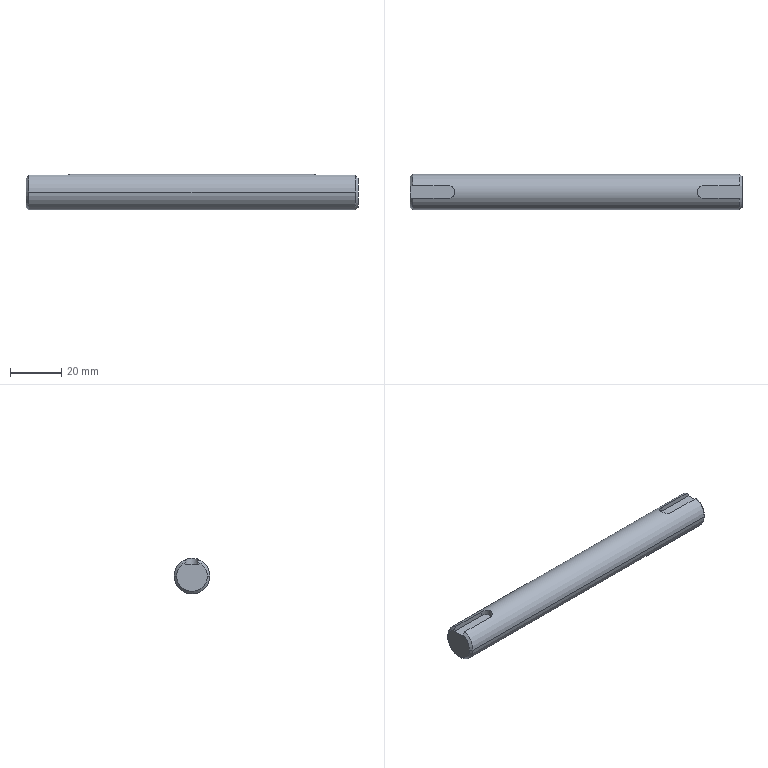Component | SolidWorks | DriveAxis-1 | 1 solid | 18 faces | box 130 x 14 x 14 mm | volume 19610 mm3 | plane 8 | cone 6 | cylinder 4 | commonest cylinder face diameters 14 x2 5 x2
build123d program:
from build123d import *

# Parameters (mm, degrees)
SKETCH1_R           = 7
BOSS_EXTRUDE1_DEPTH = 130
CHAMFER1_SIZE       = 1
CUT_EXTRUDE1_DEPTH  = 2.3


with BuildPart() as part:
    # Sketch1 → Boss-Extrude1 (new body)
    with BuildSketch(Plane(origin=(0, 0, 0), x_dir=(1, 0, 0), z_dir=(0, 1, 0))):
        with Locations(Location((0, 0, 0), (0, 0, 270))):
            Circle(SKETCH1_R)
    extrude(amount=BOSS_EXTRUDE1_DEPTH)

    # Chamfer1
    chamfer1_edges = [part.edges().sort_by_distance(p)[0] for p in [
        (0, 0, -7),
        (0, 130, -7),
    ]]
    chamfer(chamfer1_edges, length=CHAMFER1_SIZE)

    # Sketch2 → Cut-Extrude1 (cut)
    with BuildSketch(Plane.ZY.offset(7)):
        with BuildLine():
            Line((-2.5, 0), (-2.5, 15))
            ThreePointArc((-2.5, 15), (0, 17.5), (2.5, 15))
            Line((2.5, 15), (2.5, 0))
            ThreePointArc((2.5, 0), (0, -2.5), (-2.5, 0))
        make_face()
    cut_extrude1 = extrude(amount=-CUT_EXTRUDE1_DEPTH, mode=Mode.SUBTRACT)

    # Mirror1: Cut-Extrude1 across plane
    add(cut_extrude1.mirror(Plane(origin=(0, 65, 0), x_dir=(0, 0, 1), z_dir=(0, -1, 0))), mode=Mode.SUBTRACT)


solid = part.part

# Placed as in the assembly
solid = solid.moved(Location((15.629, -347.9, 460), (90, 0, -90)))
STEP:
#1=COLOUR_RGB('',0.7922,0.8196,0.9333);
#2=FILL_AREA_STYLE_COLOUR('',#1);
#3=FILL_AREA_STYLE('',(#2));
#4=SURFACE_STYLE_FILL_AREA(#3);
#5=SURFACE_SIDE_STYLE('',(#4));
#6=SURFACE_STYLE_USAGE(.BOTH.,#5);
#7=PRESENTATION_STYLE_ASSIGNMENT((#6));
#8=CARTESIAN_POINT('',(0.6153,-13.461,18.11));
#9=VERTEX_POINT('',#8);
#10=CARTESIAN_POINT('',(0.6153,-13.933,18.11));
#11=VERTEX_POINT('',#10);
#12=CARTESIAN_POINT('',(0.6153,-13.697,18.11));
#13=DIRECTION('',(-1.,0.,0.));
#14=DIRECTION('',(0.,-1.,0.));
#15=AXIS2_PLACEMENT_3D('',#12,#13,#14);
#16=CIRCLE('',#15,0.2362);
#17=EDGE_CURVE('',#9,#11,#16,.T.);
#18=ORIENTED_EDGE('',*,*,#17,.F.);
#19=CARTESIAN_POINT('',(0.6547,-13.421,18.11));
#20=VERTEX_POINT('',#19);
#21=CARTESIAN_POINT('',(0.6547,-13.421,18.11));
#22=DIRECTION('',(0.7071,0.7071,0.));
#23=VECTOR('',#22,39.37);
#24=LINE('',#21,#23);
#25=EDGE_CURVE('',#9,#20,#24,.T.);
#26=ORIENTED_EDGE('',*,*,#25,.T.);
#27=CARTESIAN_POINT('',(0.6547,-13.972,18.11));
#28=VERTEX_POINT('',#27);
#29=CARTESIAN_POINT('',(0.6547,-13.697,18.11));
#30=DIRECTION('',(1.,-0.,-0.));
#31=DIRECTION('',(0.,-1.,0.));
#32=AXIS2_PLACEMENT_3D('',#29,#30,#31);
#33=CIRCLE('',#32,0.2756);
#34=EDGE_CURVE('',#28,#20,#33,.T.);
#35=ORIENTED_EDGE('',*,*,#34,.F.);
#36=CARTESIAN_POINT('',(0.6547,-13.972,18.11));
#37=DIRECTION('',(0.7071,-0.7071,-0.));
#38=VECTOR('',#37,39.37);
#39=LINE('',#36,#38);
#40=EDGE_CURVE('',#11,#28,#39,.T.);
#41=ORIENTED_EDGE('',*,*,#40,.F.);
#42=EDGE_LOOP('',(#18,#26,#35,#41));
#43=FACE_OUTER_BOUND('',#42,.T.);
#44=CARTESIAN_POINT('',(0.6547,-13.697,18.11));
#45=DIRECTION('',(1.,-0.,-0.));
#46=DIRECTION('',(0.,-1.,0.));
#47=AXIS2_PLACEMENT_3D('',#44,#45,#46);
#48=CONICAL_SURFACE('',#47,0.2756,0.7854);
#49=ADVANCED_FACE('',(#43),#48,.T.);
#50=CARTESIAN_POINT('',(0.6153,-13.795,18.325));
#51=VERTEX_POINT('',#50);
#52=CARTESIAN_POINT('',(0.6153,-13.697,18.11));
#53=DIRECTION('',(-1.,0.,0.));
#54=DIRECTION('',(0.,-1.,0.));
#55=AXIS2_PLACEMENT_3D('',#52,#53,#54);
#56=CIRCLE('',#55,0.2362);
#57=EDGE_CURVE('',#11,#51,#56,.T.);
#58=ORIENTED_EDGE('',*,*,#57,.F.);
#59=ORIENTED_EDGE('',*,*,#40,.T.);
#60=CARTESIAN_POINT('',(0.6547,-13.795,18.368));
#61=VERTEX_POINT('',#60);
#62=CARTESIAN_POINT('',(0.6547,-13.697,18.11));
#63=DIRECTION('',(1.,-0.,-0.));
#64=DIRECTION('',(0.,-1.,0.));
#65=AXIS2_PLACEMENT_3D('',#62,#63,#64);
#66=CIRCLE('',#65,0.2756);
#67=EDGE_CURVE('',#61,#28,#66,.T.);
#68=ORIENTED_EDGE('',*,*,#67,.F.);
#69=CARTESIAN_POINT('',(0.6153,-13.795,18.325));
#70=CARTESIAN_POINT('',(0.6283,-13.795,18.339));
#71=CARTESIAN_POINT('',(0.6415,-13.795,18.354));
#72=CARTESIAN_POINT('',(0.6547,-13.795,18.368));
#73=B_SPLINE_CURVE_WITH_KNOTS('',3,(#69,#70,#71,#72),.UNSPECIFIED.,.F.,.F.,(4,4),(0.003923,0.005397),.UNSPECIFIED.);
#74=EDGE_CURVE('',#51,#61,#73,.T.);
#75=ORIENTED_EDGE('',*,*,#74,.F.);
#76=EDGE_LOOP('',(#58,#59,#68,#75));
#77=FACE_OUTER_BOUND('',#76,.T.);
#78=CARTESIAN_POINT('',(0.6547,-13.697,18.11));
#79=DIRECTION('',(1.,-0.,-0.));
#80=DIRECTION('',(0.,-1.,0.));
#81=AXIS2_PLACEMENT_3D('',#78,#79,#80);
#82=CONICAL_SURFACE('',#81,0.2756,0.7854);
#83=ADVANCED_FACE('',(#77),#82,.T.);
#84=CARTESIAN_POINT('',(5.733,-13.933,18.11));
#85=VERTEX_POINT('',#84);
#86=CARTESIAN_POINT('',(5.733,-13.461,18.11));
#87=VERTEX_POINT('',#86);
#88=CARTESIAN_POINT('',(5.733,-13.697,18.11));
#89=DIRECTION('',(1.,-0.,-0.));
#90=DIRECTION('',(0.,-1.,0.));
#91=AXIS2_PLACEMENT_3D('',#88,#89,#90);
#92=CIRCLE('',#91,0.2362);
#93=EDGE_CURVE('',#85,#87,#92,.T.);
#94=ORIENTED_EDGE('',*,*,#93,.F.);
#95=CARTESIAN_POINT('',(5.694,-13.972,18.11));
#96=VERTEX_POINT('',#95);
#97=CARTESIAN_POINT('',(5.733,-13.933,18.11));
#98=DIRECTION('',(-0.7071,-0.7071,-0.));
#99=VECTOR('',#98,39.37);
#100=LINE('',#97,#99);
#101=EDGE_CURVE('',#85,#96,#100,.T.);
#102=ORIENTED_EDGE('',*,*,#101,.T.);
#103=CARTESIAN_POINT('',(5.694,-13.421,18.11));
#104=VERTEX_POINT('',#103);
#105=CARTESIAN_POINT('',(5.694,-13.697,18.11));
#106=DIRECTION('',(-1.,0.,0.));
#107=DIRECTION('',(0.,-1.,-0.));
#108=AXIS2_PLACEMENT_3D('',#105,#106,#107);
#109=CIRCLE('',#108,0.2756);
#110=EDGE_CURVE('',#104,#96,#109,.T.);
#111=ORIENTED_EDGE('',*,*,#110,.F.);
#112=CARTESIAN_POINT('',(5.733,-13.461,18.11));
#113=DIRECTION('',(-0.7071,0.7071,0.));
#114=VECTOR('',#113,39.37);
#115=LINE('',#112,#114);
#116=EDGE_CURVE('',#87,#104,#115,.T.);
#117=ORIENTED_EDGE('',*,*,#116,.F.);
#118=EDGE_LOOP('',(#94,#102,#111,#117));
#119=FACE_OUTER_BOUND('',#118,.T.);
#120=CARTESIAN_POINT('',(5.733,-13.697,18.11));
#121=DIRECTION('',(-1.,0.,0.));
#122=DIRECTION('',(0.,1.,0.));
#123=AXIS2_PLACEMENT_3D('',#120,#121,#122);
#124=CONICAL_SURFACE('',#123,0.2362,0.7854);
#125=ADVANCED_FACE('',(#119),#124,.T.);
#126=CARTESIAN_POINT('',(5.733,-13.598,18.325));
#127=VERTEX_POINT('',#126);
#128=CARTESIAN_POINT('',(5.733,-13.697,18.11));
#129=DIRECTION('',(1.,-0.,-0.));
#130=DIRECTION('',(0.,-1.,0.));
#131=AXIS2_PLACEMENT_3D('',#128,#129,#130);
#132=CIRCLE('',#131,0.2362);
#133=EDGE_CURVE('',#87,#127,#132,.T.);
#134=ORIENTED_EDGE('',*,*,#133,.F.);
#135=ORIENTED_EDGE('',*,*,#116,.T.);
#136=CARTESIAN_POINT('',(5.694,-13.598,18.368));
#137=VERTEX_POINT('',#136);
#138=CARTESIAN_POINT('',(5.694,-13.697,18.11));
#139=DIRECTION('',(-1.,0.,0.));
#140=DIRECTION('',(0.,-1.,-0.));
#141=AXIS2_PLACEMENT_3D('',#138,#139,#140);
#142=CIRCLE('',#141,0.2756);
#143=EDGE_CURVE('',#137,#104,#142,.T.);
#144=ORIENTED_EDGE('',*,*,#143,.F.);
#145=CARTESIAN_POINT('',(5.694,-13.598,18.368));
#146=CARTESIAN_POINT('',(5.707,-13.598,18.354));
#147=CARTESIAN_POINT('',(5.72,-13.598,18.339));
#148=CARTESIAN_POINT('',(5.733,-13.598,18.325));
#149=B_SPLINE_CURVE_WITH_KNOTS('',3,(#145,#146,#147,#148),.UNSPECIFIED.,.F.,.F.,(4,4),(0.003636,0.005111),.UNSPECIFIED.);
#150=EDGE_CURVE('',#137,#127,#149,.T.);
#151=ORIENTED_EDGE('',*,*,#150,.T.);
#152=EDGE_LOOP('',(#134,#135,#144,#151));
#153=FACE_OUTER_BOUND('',#152,.T.);
#154=CARTESIAN_POINT('',(5.733,-13.697,18.11));
#155=DIRECTION('',(-1.,0.,0.));
#156=DIRECTION('',(0.,1.,0.));
#157=AXIS2_PLACEMENT_3D('',#154,#155,#156);
#158=CONICAL_SURFACE('',#157,0.2362,0.7854);
#159=ADVANCED_FACE('',(#153),#158,.T.);
#160=ORIENTED_EDGE('',*,*,#110,.T.);
#161=CARTESIAN_POINT('',(5.733,-13.972,18.11));
#162=DIRECTION('',(-1.,0.,0.));
#163=VECTOR('',#162,39.37);
#164=LINE('',#161,#163);
#165=EDGE_CURVE('',#96,#28,#164,.T.);
#166=ORIENTED_EDGE('',*,*,#165,.T.);
#167=ORIENTED_EDGE('',*,*,#34,.T.);
#168=CARTESIAN_POINT('',(5.733,-13.421,18.11));
#169=DIRECTION('',(-1.,0.,0.));
#170=VECTOR('',#169,39.37);
#171=LINE('',#168,#170);
#172=EDGE_CURVE('',#104,#20,#171,.T.);
#173=ORIENTED_EDGE('',*,*,#172,.F.);
#174=EDGE_LOOP('',(#160,#166,#167,#173));
#175=FACE_OUTER_BOUND('',#174,.T.);
#176=CARTESIAN_POINT('',(5.733,-13.697,18.11));
#177=DIRECTION('',(-1.,0.,0.));
#178=DIRECTION('',(0.,1.,0.));
#179=AXIS2_PLACEMENT_3D('',#176,#177,#178);
#180=CYLINDRICAL_SURFACE('',#179,0.2756);
#181=ADVANCED_FACE('',(#175),#180,.T.);
#182=ORIENTED_EDGE('',*,*,#165,.F.);
#183=CARTESIAN_POINT('',(5.694,-13.795,18.368));
#184=VERTEX_POINT('',#183);
#185=CARTESIAN_POINT('',(5.694,-13.697,18.11));
#186=DIRECTION('',(-1.,0.,0.));
#187=DIRECTION('',(0.,-1.,0.));
#188=AXIS2_PLACEMENT_3D('',#185,#186,#187);
#189=CIRCLE('',#188,0.2756);
#190=EDGE_CURVE('',#96,#184,#189,.T.);
#191=ORIENTED_EDGE('',*,*,#190,.T.);
#192=CARTESIAN_POINT('',(5.143,-13.795,18.368));
#193=VERTEX_POINT('',#192);
#194=CARTESIAN_POINT('',(5.733,-13.795,18.368));
#195=DIRECTION('',(1.,-0.,-0.));
#196=VECTOR('',#195,39.37);
#197=LINE('',#194,#196);
#198=EDGE_CURVE('',#193,#184,#197,.T.);
#199=ORIENTED_EDGE('',*,*,#198,.F.);
#200=CARTESIAN_POINT('',(5.143,-13.598,18.368));
#201=VERTEX_POINT('',#200);
#202=CARTESIAN_POINT('',(5.143,-13.598,18.368));
#203=CARTESIAN_POINT('',(5.136,-13.598,18.368));
#204=CARTESIAN_POINT('',(5.13,-13.599,18.368));
#205=CARTESIAN_POINT('',(5.117,-13.602,18.369));
#206=CARTESIAN_POINT('',(5.111,-13.604,18.37));
#207=CARTESIAN_POINT('',(5.099,-13.608,18.371));
#208=CARTESIAN_POINT('',(5.093,-13.612,18.372));
#209=CARTESIAN_POINT('',(5.083,-13.619,18.375));
#210=CARTESIAN_POINT('',(5.078,-13.623,18.376));
#211=CARTESIAN_POINT('',(5.064,-13.636,18.379));
#212=CARTESIAN_POINT('',(5.057,-13.647,18.382));
#213=CARTESIAN_POINT('',(5.05,-13.665,18.384));
#214=CARTESIAN_POINT('',(5.048,-13.671,18.385));
#215=CARTESIAN_POINT('',(5.045,-13.684,18.386));
#216=CARTESIAN_POINT('',(5.044,-13.69,18.386));
#217=CARTESIAN_POINT('',(5.044,-13.703,18.386));
#218=CARTESIAN_POINT('',(5.045,-13.71,18.386));
#219=CARTESIAN_POINT('',(5.048,-13.722,18.385));
#220=CARTESIAN_POINT('',(5.05,-13.729,18.384));
#221=CARTESIAN_POINT('',(5.054,-13.741,18.382));
#222=CARTESIAN_POINT('',(5.058,-13.746,18.381));
#223=CARTESIAN_POINT('',(5.065,-13.757,18.379));
#224=CARTESIAN_POINT('',(5.069,-13.762,18.378));
#225=CARTESIAN_POINT('',(5.078,-13.771,18.376));
#226=CARTESIAN_POINT('',(5.083,-13.775,18.375));
#227=CARTESIAN_POINT('',(5.093,-13.782,18.372));
#228=CARTESIAN_POINT('',(5.099,-13.785,18.371));
#229=CARTESIAN_POINT('',(5.111,-13.79,18.37));
#230=CARTESIAN_POINT('',(5.117,-13.792,18.369));
#231=CARTESIAN_POINT('',(5.13,-13.795,18.368));
#232=CARTESIAN_POINT('',(5.136,-13.795,18.368));
#233=CARTESIAN_POINT('',(5.143,-13.795,18.368));
#234=B_SPLINE_CURVE_WITH_KNOTS('',3,(#202,#203,#204,#205,#206,#207,#208,#209,#210,#211,#212,#213,#214,#215,#216,#217,#218,#219,#220,#221,#222,#223,#224,#225,#226,#227,#228,#229,#230,#231,#232,#233),.UNSPECIFIED.,.F.,.F.,(4,2,2,2,2,2,2,2,2,2,2,2,2,2,2,4),(0.,0.0004924,0.0009848,0.001477,0.00197,0.002954,0.003447,0.003939,0.004432,0.004924,0.005416,0.005909,0.006401,0.006894,0.007386,0.007878),.UNSPECIFIED.);
#235=EDGE_CURVE('',#201,#193,#234,.T.);
#236=ORIENTED_EDGE('',*,*,#235,.F.);
#237=CARTESIAN_POINT('',(5.733,-13.598,18.368));
#238=DIRECTION('',(-1.,0.,0.));
#239=VECTOR('',#238,39.37);
#240=LINE('',#237,#239);
#241=EDGE_CURVE('',#137,#201,#240,.T.);
#242=ORIENTED_EDGE('',*,*,#241,.F.);
#243=ORIENTED_EDGE('',*,*,#143,.T.);
#244=ORIENTED_EDGE('',*,*,#172,.T.);
#245=CARTESIAN_POINT('',(0.6547,-13.598,18.368));
#246=VERTEX_POINT('',#245);
#247=CARTESIAN_POINT('',(0.6547,-13.697,18.11));
#248=DIRECTION('',(1.,-0.,-0.));
#249=DIRECTION('',(0.,-1.,0.));
#250=AXIS2_PLACEMENT_3D('',#247,#248,#249);
#251=CIRCLE('',#250,0.2756);
#252=EDGE_CURVE('',#20,#246,#251,.T.);
#253=ORIENTED_EDGE('',*,*,#252,.T.);
#254=CARTESIAN_POINT('',(1.206,-13.598,18.368));
#255=VERTEX_POINT('',#254);
#256=CARTESIAN_POINT('',(5.733,-13.598,18.368));
#257=DIRECTION('',(1.,-0.,-0.));
#258=VECTOR('',#257,39.37);
#259=LINE('',#256,#258);
#260=EDGE_CURVE('',#246,#255,#259,.T.);
#261=ORIENTED_EDGE('',*,*,#260,.T.);
#262=CARTESIAN_POINT('',(1.206,-13.795,18.368));
#263=VERTEX_POINT('',#262);
#264=CARTESIAN_POINT('',(1.206,-13.598,18.368));
#265=CARTESIAN_POINT('',(1.212,-13.598,18.368));
#266=CARTESIAN_POINT('',(1.219,-13.599,18.368));
#267=CARTESIAN_POINT('',(1.232,-13.602,18.369));
#268=CARTESIAN_POINT('',(1.238,-13.604,18.37));
#269=CARTESIAN_POINT('',(1.25,-13.608,18.371));
#270=CARTESIAN_POINT('',(1.255,-13.612,18.372));
#271=CARTESIAN_POINT('',(1.266,-13.619,18.375));
#272=CARTESIAN_POINT('',(1.271,-13.623,18.376));
#273=CARTESIAN_POINT('',(1.284,-13.636,18.379));
#274=CARTESIAN_POINT('',(1.292,-13.647,18.382));
#275=CARTESIAN_POINT('',(1.299,-13.665,18.384));
#276=CARTESIAN_POINT('',(1.301,-13.671,18.385));
#277=CARTESIAN_POINT('',(1.304,-13.684,18.386));
#278=CARTESIAN_POINT('',(1.304,-13.69,18.386));
#279=CARTESIAN_POINT('',(1.304,-13.703,18.386));
#280=CARTESIAN_POINT('',(1.304,-13.71,18.386));
#281=CARTESIAN_POINT('',(1.301,-13.722,18.385));
#282=CARTESIAN_POINT('',(1.299,-13.729,18.384));
#283=CARTESIAN_POINT('',(1.294,-13.741,18.382));
#284=CARTESIAN_POINT('',(1.291,-13.746,18.381));
#285=CARTESIAN_POINT('',(1.284,-13.757,18.379));
#286=CARTESIAN_POINT('',(1.28,-13.762,18.378));
#287=CARTESIAN_POINT('',(1.271,-13.771,18.376));
#288=CARTESIAN_POINT('',(1.266,-13.775,18.375));
#289=CARTESIAN_POINT('',(1.255,-13.782,18.372));
#290=CARTESIAN_POINT('',(1.25,-13.785,18.371));
#291=CARTESIAN_POINT('',(1.238,-13.79,18.37));
#292=CARTESIAN_POINT('',(1.232,-13.792,18.369));
#293=CARTESIAN_POINT('',(1.219,-13.795,18.368));
#294=CARTESIAN_POINT('',(1.212,-13.795,18.368));
#295=CARTESIAN_POINT('',(1.206,-13.795,18.368));
#296=B_SPLINE_CURVE_WITH_KNOTS('',3,(#264,#265,#266,#267,#268,#269,#270,#271,#272,#273,#274,#275,#276,#277,#278,#279,#280,#281,#282,#283,#284,#285,#286,#287,#288,#289,#290,#291,#292,#293,#294,#295),.UNSPECIFIED.,.F.,.F.,(4,2,2,2,2,2,2,2,2,2,2,2,2,2,2,4),(0.,0.0004924,0.0009848,0.001477,0.00197,0.002954,0.003447,0.003939,0.004432,0.004924,0.005416,0.005909,0.006401,0.006894,0.007386,0.007878),.UNSPECIFIED.);
#297=EDGE_CURVE('',#255,#263,#296,.T.);
#298=ORIENTED_EDGE('',*,*,#297,.T.);
#299=CARTESIAN_POINT('',(5.733,-13.795,18.368));
#300=DIRECTION('',(-1.,0.,0.));
#301=VECTOR('',#300,39.37);
#302=LINE('',#299,#301);
#303=EDGE_CURVE('',#263,#61,#302,.T.);
#304=ORIENTED_EDGE('',*,*,#303,.T.);
#305=ORIENTED_EDGE('',*,*,#67,.T.);
#306=EDGE_LOOP('',(#182,#191,#199,#236,#242,#243,#244,#253,#261,#298,#304,#305));
#307=FACE_OUTER_BOUND('',#306,.T.);
#308=CARTESIAN_POINT('',(5.733,-13.697,18.11));
#309=DIRECTION('',(-1.,0.,0.));
#310=DIRECTION('',(0.,1.,0.));
#311=AXIS2_PLACEMENT_3D('',#308,#309,#310);
#312=CYLINDRICAL_SURFACE('',#311,0.2756);
#313=ADVANCED_FACE('',(#307),#312,.T.);
#314=CARTESIAN_POINT('',(5.733,-13.598,18.295));
#315=VERTEX_POINT('',#314);
#316=CARTESIAN_POINT('',(5.733,-13.795,18.295));
#317=VERTEX_POINT('',#316);
#318=CARTESIAN_POINT('',(5.733,-13.697,18.295));
#319=DIRECTION('',(-0.,-1.,-0.));
#320=VECTOR('',#319,39.37);
#321=LINE('',#318,#320);
#322=EDGE_CURVE('',#315,#317,#321,.T.);
#323=ORIENTED_EDGE('',*,*,#322,.T.);
#324=CARTESIAN_POINT('',(5.733,-13.795,18.325));
#325=VERTEX_POINT('',#324);
#326=CARTESIAN_POINT('',(5.733,-13.795,18.295));
#327=DIRECTION('',(0.,-0.,1.));
#328=VECTOR('',#327,39.37);
#329=LINE('',#326,#328);
#330=EDGE_CURVE('',#317,#325,#329,.T.);
#331=ORIENTED_EDGE('',*,*,#330,.T.);
#332=CARTESIAN_POINT('',(5.733,-13.697,18.11));
#333=DIRECTION('',(1.,-0.,-0.));
#334=DIRECTION('',(0.,-1.,0.));
#335=AXIS2_PLACEMENT_3D('',#332,#333,#334);
#336=CIRCLE('',#335,0.2362);
#337=EDGE_CURVE('',#325,#85,#336,.T.);
#338=ORIENTED_EDGE('',*,*,#337,.T.);
#339=ORIENTED_EDGE('',*,*,#93,.T.);
#340=ORIENTED_EDGE('',*,*,#133,.T.);
#341=CARTESIAN_POINT('',(5.733,-13.598,18.295));
#342=DIRECTION('',(0.,-0.,1.));
#343=VECTOR('',#342,39.37);
#344=LINE('',#341,#343);
#345=EDGE_CURVE('',#315,#127,#344,.T.);
#346=ORIENTED_EDGE('',*,*,#345,.F.);
#347=EDGE_LOOP('',(#323,#331,#338,#339,#340,#346));
#348=FACE_OUTER_BOUND('',#347,.T.);
#349=CARTESIAN_POINT('',(5.733,-13.697,18.11));
#350=DIRECTION('',(1.,-0.,-0.));
#351=DIRECTION('',(-0.,-1.,-0.));
#352=AXIS2_PLACEMENT_3D('',#349,#350,#351);
#353=PLANE('',#352);
#354=ADVANCED_FACE('',(#348),#353,.T.);
#355=ORIENTED_EDGE('',*,*,#101,.F.);
#356=ORIENTED_EDGE('',*,*,#337,.F.);
#357=CARTESIAN_POINT('',(5.733,-13.795,18.325));
#358=CARTESIAN_POINT('',(5.72,-13.795,18.339));
#359=CARTESIAN_POINT('',(5.707,-13.795,18.354));
#360=CARTESIAN_POINT('',(5.694,-13.795,18.368));
#361=B_SPLINE_CURVE_WITH_KNOTS('',3,(#357,#358,#359,#360),.UNSPECIFIED.,.F.,.F.,(4,4),(0.003923,0.005397),.UNSPECIFIED.);
#362=EDGE_CURVE('',#325,#184,#361,.T.);
#363=ORIENTED_EDGE('',*,*,#362,.T.);
#364=ORIENTED_EDGE('',*,*,#190,.F.);
#365=EDGE_LOOP('',(#355,#356,#363,#364));
#366=FACE_OUTER_BOUND('',#365,.T.);
#367=CARTESIAN_POINT('',(5.733,-13.697,18.11));
#368=DIRECTION('',(-1.,0.,0.));
#369=DIRECTION('',(0.,1.,0.));
#370=AXIS2_PLACEMENT_3D('',#367,#368,#369);
#371=CONICAL_SURFACE('',#370,0.2362,0.7854);
#372=ADVANCED_FACE('',(#366),#371,.T.);
#373=CARTESIAN_POINT('',(0.6153,-13.598,18.295));
#374=VERTEX_POINT('',#373);
#375=CARTESIAN_POINT('',(0.6153,-13.795,18.295));
#376=VERTEX_POINT('',#375);
#377=CARTESIAN_POINT('',(0.6153,-13.697,18.295));
#378=DIRECTION('',(-0.,-1.,-0.));
#379=VECTOR('',#378,39.37);
#380=LINE('',#377,#379);
#381=EDGE_CURVE('',#374,#376,#380,.T.);
#382=ORIENTED_EDGE('',*,*,#381,.F.);
#383=CARTESIAN_POINT('',(0.6153,-13.598,18.325));
#384=VERTEX_POINT('',#383);
#385=CARTESIAN_POINT('',(0.6153,-13.598,18.295));
#386=DIRECTION('',(0.,-0.,1.));
#387=VECTOR('',#386,39.37);
#388=LINE('',#385,#387);
#389=EDGE_CURVE('',#374,#384,#388,.T.);
#390=ORIENTED_EDGE('',*,*,#389,.T.);
#391=CARTESIAN_POINT('',(0.6153,-13.697,18.11));
#392=DIRECTION('',(-1.,0.,0.));
#393=DIRECTION('',(0.,-1.,0.));
#394=AXIS2_PLACEMENT_3D('',#391,#392,#393);
#395=CIRCLE('',#394,0.2362);
#396=EDGE_CURVE('',#384,#9,#395,.T.);
#397=ORIENTED_EDGE('',*,*,#396,.T.);
#398=ORIENTED_EDGE('',*,*,#17,.T.);
#399=ORIENTED_EDGE('',*,*,#57,.T.);
#400=CARTESIAN_POINT('',(0.6153,-13.795,18.295));
#401=DIRECTION('',(0.,-0.,1.));
#402=VECTOR('',#401,39.37);
#403=LINE('',#400,#402);
#404=EDGE_CURVE('',#376,#51,#403,.T.);
#405=ORIENTED_EDGE('',*,*,#404,.F.);
#406=EDGE_LOOP('',(#382,#390,#397,#398,#399,#405));
#407=FACE_OUTER_BOUND('',#406,.T.);
#408=CARTESIAN_POINT('',(0.6153,-13.697,18.11));
#409=DIRECTION('',(1.,-0.,-0.));
#410=DIRECTION('',(-0.,-1.,-0.));
#411=AXIS2_PLACEMENT_3D('',#408,#409,#410);
#412=PLANE('',#411);
#413=ADVANCED_FACE('',(#407),#412,.F.);
#414=ORIENTED_EDGE('',*,*,#25,.F.);
#415=ORIENTED_EDGE('',*,*,#396,.F.);
#416=CARTESIAN_POINT('',(0.6547,-13.598,18.368));
#417=CARTESIAN_POINT('',(0.6415,-13.598,18.354));
#418=CARTESIAN_POINT('',(0.6283,-13.598,18.339));
#419=CARTESIAN_POINT('',(0.6153,-13.598,18.325));
#420=B_SPLINE_CURVE_WITH_KNOTS('',3,(#416,#417,#418,#419),.UNSPECIFIED.,.F.,.F.,(4,4),(0.003636,0.005111),.UNSPECIFIED.);
#421=EDGE_CURVE('',#246,#384,#420,.T.);
#422=ORIENTED_EDGE('',*,*,#421,.F.);
#423=ORIENTED_EDGE('',*,*,#252,.F.);
#424=EDGE_LOOP('',(#414,#415,#422,#423));
#425=FACE_OUTER_BOUND('',#424,.T.);
#426=CARTESIAN_POINT('',(0.6547,-13.697,18.11));
#427=DIRECTION('',(1.,-0.,-0.));
#428=DIRECTION('',(0.,-1.,0.));
#429=AXIS2_PLACEMENT_3D('',#426,#427,#428);
#430=CONICAL_SURFACE('',#429,0.2756,0.7854);
#431=ADVANCED_FACE('',(#425),#430,.T.);
#432=CARTESIAN_POINT('',(1.206,-13.598,18.295));
#433=VERTEX_POINT('',#432);
#434=CARTESIAN_POINT('',(1.206,-13.598,18.295));
#435=DIRECTION('',(0.,-0.,1.));
#436=VECTOR('',#435,39.37);
#437=LINE('',#434,#436);
#438=EDGE_CURVE('',#433,#255,#437,.T.);
#439=ORIENTED_EDGE('',*,*,#438,.F.);
#440=CARTESIAN_POINT('',(1.206,-13.795,18.295));
#441=VERTEX_POINT('',#440);
#442=CARTESIAN_POINT('',(1.206,-13.697,18.295));
#443=DIRECTION('',(0.,-0.,1.));
#444=DIRECTION('',(0.,-1.,0.));
#445=AXIS2_PLACEMENT_3D('',#442,#443,#444);
#446=CIRCLE('',#445,0.09843);
#447=EDGE_CURVE('',#441,#433,#446,.T.);
#448=ORIENTED_EDGE('',*,*,#447,.F.);
#449=CARTESIAN_POINT('',(1.206,-13.795,18.295));
#450=DIRECTION('',(0.,-0.,1.));
#451=VECTOR('',#450,39.37);
#452=LINE('',#449,#451);
#453=EDGE_CURVE('',#441,#263,#452,.T.);
#454=ORIENTED_EDGE('',*,*,#453,.T.);
#455=ORIENTED_EDGE('',*,*,#297,.F.);
#456=EDGE_LOOP('',(#439,#448,#454,#455));
#457=FACE_OUTER_BOUND('',#456,.T.);
#458=CARTESIAN_POINT('',(1.206,-13.697,18.295));
#459=DIRECTION('',(0.,-0.,1.));
#460=DIRECTION('',(0.,-1.,0.));
#461=AXIS2_PLACEMENT_3D('',#458,#459,#460);
#462=CYLINDRICAL_SURFACE('',#461,0.09843);
#463=ADVANCED_FACE('',(#457),#462,.F.);
#464=ORIENTED_EDGE('',*,*,#381,.T.);
#465=CARTESIAN_POINT('',(0.6153,-13.795,18.295));
#466=DIRECTION('',(1.,-0.,-0.));
#467=VECTOR('',#466,39.37);
#468=LINE('',#465,#467);
#469=EDGE_CURVE('',#376,#441,#468,.T.);
#470=ORIENTED_EDGE('',*,*,#469,.T.);
#471=ORIENTED_EDGE('',*,*,#447,.T.);
#472=CARTESIAN_POINT('',(0.6153,-13.598,18.295));
#473=DIRECTION('',(-1.,0.,0.));
#474=VECTOR('',#473,39.37);
#475=LINE('',#472,#474);
#476=EDGE_CURVE('',#433,#374,#475,.T.);
#477=ORIENTED_EDGE('',*,*,#476,.T.);
#478=EDGE_LOOP('',(#464,#470,#471,#477));
#479=FACE_OUTER_BOUND('',#478,.T.);
#480=CARTESIAN_POINT('',(0.6153,-13.697,18.295));
#481=DIRECTION('',(0.,-0.,1.));
#482=DIRECTION('',(-0.,-1.,-0.));
#483=AXIS2_PLACEMENT_3D('',#480,#481,#482);
#484=PLANE('',#483);
#485=ADVANCED_FACE('',(#479),#484,.T.);
#486=ORIENTED_EDGE('',*,*,#421,.T.);
#487=ORIENTED_EDGE('',*,*,#389,.F.);
#488=ORIENTED_EDGE('',*,*,#476,.F.);
#489=ORIENTED_EDGE('',*,*,#438,.T.);
#490=ORIENTED_EDGE('',*,*,#260,.F.);
#491=EDGE_LOOP('',(#486,#487,#488,#489,#490));
#492=FACE_OUTER_BOUND('',#491,.T.);
#493=CARTESIAN_POINT('',(0.6153,-13.598,18.295));
#494=DIRECTION('',(0.,1.,0.));
#495=DIRECTION('',(0.,-0.,1.));
#496=AXIS2_PLACEMENT_3D('',#493,#494,#495);
#497=PLANE('',#496);
#498=ADVANCED_FACE('',(#492),#497,.F.);
#499=ORIENTED_EDGE('',*,*,#453,.F.);
#500=ORIENTED_EDGE('',*,*,#469,.F.);
#501=ORIENTED_EDGE('',*,*,#404,.T.);
#502=ORIENTED_EDGE('',*,*,#74,.T.);
#503=ORIENTED_EDGE('',*,*,#303,.F.);
#504=EDGE_LOOP('',(#499,#500,#501,#502,#503));
#505=FACE_OUTER_BOUND('',#504,.T.);
#506=CARTESIAN_POINT('',(0.6153,-13.795,18.295));
#507=DIRECTION('',(-0.,-1.,-0.));
#508=DIRECTION('',(-0.,0.,-1.));
#509=AXIS2_PLACEMENT_3D('',#506,#507,#508);
#510=PLANE('',#509);
#511=ADVANCED_FACE('',(#505),#510,.F.);
#512=CARTESIAN_POINT('',(5.143,-13.598,18.295));
#513=VERTEX_POINT('',#512);
#514=CARTESIAN_POINT('',(5.143,-13.598,18.295));
#515=DIRECTION('',(0.,-0.,1.));
#516=VECTOR('',#515,39.37);
#517=LINE('',#514,#516);
#518=EDGE_CURVE('',#513,#201,#517,.T.);
#519=ORIENTED_EDGE('',*,*,#518,.T.);
#520=ORIENTED_EDGE('',*,*,#235,.T.);
#521=CARTESIAN_POINT('',(5.143,-13.795,18.295));
#522=VERTEX_POINT('',#521);
#523=CARTESIAN_POINT('',(5.143,-13.795,18.295));
#524=DIRECTION('',(0.,-0.,1.));
#525=VECTOR('',#524,39.37);
#526=LINE('',#523,#525);
#527=EDGE_CURVE('',#522,#193,#526,.T.);
#528=ORIENTED_EDGE('',*,*,#527,.F.);
#529=CARTESIAN_POINT('',(5.143,-13.697,18.295));
#530=DIRECTION('',(-0.,0.,-1.));
#531=DIRECTION('',(0.,-1.,0.));
#532=AXIS2_PLACEMENT_3D('',#529,#530,#531);
#533=CIRCLE('',#532,0.09843);
#534=EDGE_CURVE('',#522,#513,#533,.T.);
#535=ORIENTED_EDGE('',*,*,#534,.T.);
#536=EDGE_LOOP('',(#519,#520,#528,#535));
#537=FACE_OUTER_BOUND('',#536,.T.);
#538=CARTESIAN_POINT('',(5.143,-13.697,18.295));
#539=DIRECTION('',(0.,-0.,1.));
#540=DIRECTION('',(0.,-1.,0.));
#541=AXIS2_PLACEMENT_3D('',#538,#539,#540);
#542=CYLINDRICAL_SURFACE('',#541,0.09843);
#543=ADVANCED_FACE('',(#537),#542,.F.);
#544=ORIENTED_EDGE('',*,*,#198,.T.);
#545=ORIENTED_EDGE('',*,*,#362,.F.);
#546=ORIENTED_EDGE('',*,*,#330,.F.);
#547=CARTESIAN_POINT('',(5.733,-13.795,18.295));
#548=DIRECTION('',(-1.,0.,0.));
#549=VECTOR('',#548,39.37);
#550=LINE('',#547,#549);
#551=EDGE_CURVE('',#317,#522,#550,.T.);
#552=ORIENTED_EDGE('',*,*,#551,.T.);
#553=ORIENTED_EDGE('',*,*,#527,.T.);
#554=EDGE_LOOP('',(#544,#545,#546,#552,#553));
#555=FACE_OUTER_BOUND('',#554,.T.);
#556=CARTESIAN_POINT('',(5.733,-13.795,18.295));
#557=DIRECTION('',(0.,1.,0.));
#558=DIRECTION('',(0.,-0.,1.));
#559=AXIS2_PLACEMENT_3D('',#556,#557,#558);
#560=PLANE('',#559);
#561=ADVANCED_FACE('',(#555),#560,.T.);
#562=ORIENTED_EDGE('',*,*,#241,.T.);
#563=ORIENTED_EDGE('',*,*,#518,.F.);
#564=CARTESIAN_POINT('',(5.733,-13.598,18.295));
#565=DIRECTION('',(1.,-0.,-0.));
#566=VECTOR('',#565,39.37);
#567=LINE('',#564,#566);
#568=EDGE_CURVE('',#513,#315,#567,.T.);
#569=ORIENTED_EDGE('',*,*,#568,.T.);
#570=ORIENTED_EDGE('',*,*,#345,.T.);
#571=ORIENTED_EDGE('',*,*,#150,.F.);
#572=EDGE_LOOP('',(#562,#563,#569,#570,#571));
#573=FACE_OUTER_BOUND('',#572,.T.);
#574=CARTESIAN_POINT('',(5.733,-13.598,18.295));
#575=DIRECTION('',(-0.,-1.,-0.));
#576=DIRECTION('',(-0.,0.,-1.));
#577=AXIS2_PLACEMENT_3D('',#574,#575,#576);
#578=PLANE('',#577);
#579=ADVANCED_FACE('',(#573),#578,.T.);
#580=ORIENTED_EDGE('',*,*,#568,.F.);
#581=ORIENTED_EDGE('',*,*,#534,.F.);
#582=ORIENTED_EDGE('',*,*,#551,.F.);
#583=ORIENTED_EDGE('',*,*,#322,.F.);
#584=EDGE_LOOP('',(#580,#581,#582,#583));
#585=FACE_OUTER_BOUND('',#584,.T.);
#586=CARTESIAN_POINT('',(5.733,-13.697,18.295));
#587=DIRECTION('',(0.,-0.,1.));
#588=DIRECTION('',(-0.,-1.,-0.));
#589=AXIS2_PLACEMENT_3D('',#586,#587,#588);
#590=PLANE('',#589);
#591=ADVANCED_FACE('',(#585),#590,.T.);
#592=CLOSED_SHELL('',(#49,#83,#125,#159,#181,#313,#354,#372,#413,#431,#463,#485,#498,#511,#543,#561,#579,#591));
#593=MANIFOLD_SOLID_BREP('',#592);
#594=STYLED_ITEM('',(#7),#593);
#595=PRESENTATION_LAYER_ASSIGNMENT('','',(#594));
#596=(LENGTH_UNIT()NAMED_UNIT(*)SI_UNIT($,.METRE.));
#597=LENGTH_MEASURE_WITH_UNIT(LENGTH_MEASURE(0.0254),#596);
#598=DIMENSIONAL_EXPONENTS(1.,0.,0.,0.,0.,0.,0.);
#599=(CONVERSION_BASED_UNIT('',#597)LENGTH_UNIT()NAMED_UNIT(#598));
#600=UNCERTAINTY_MEASURE_WITH_UNIT(LENGTH_MEASURE(0.00001),#599,'','');
#601=(NAMED_UNIT(*)PLANE_ANGLE_UNIT()SI_UNIT($,.RADIAN.));
#602=(NAMED_UNIT(*)SI_UNIT($,.STERADIAN.)SOLID_ANGLE_UNIT());
#603=(GEOMETRIC_REPRESENTATION_CONTEXT(3)GLOBAL_UNCERTAINTY_ASSIGNED_CONTEXT((#600))GLOBAL_UNIT_ASSIGNED_CONTEXT((#599,#601,#602))REPRESENTATION_CONTEXT('',''));
#604=MECHANICAL_DESIGN_GEOMETRIC_PRESENTATION_REPRESENTATION('',(#594),#603);
#605=CARTESIAN_POINT('',(0.,0.,0.));
#606=DIRECTION('',(0.,0.,1.));
#607=DIRECTION('',(1.,0.,0.));
#608=AXIS2_PLACEMENT_3D('',#605,#606,#607);
#609=(LENGTH_UNIT()NAMED_UNIT(*)SI_UNIT($,.METRE.));
#610=LENGTH_MEASURE_WITH_UNIT(LENGTH_MEASURE(0.0254),#609);
#611=DIMENSIONAL_EXPONENTS(1.,0.,0.,0.,0.,0.,0.);
#612=(CONVERSION_BASED_UNIT('',#610)LENGTH_UNIT()NAMED_UNIT(#611));
#613=UNCERTAINTY_MEASURE_WITH_UNIT(LENGTH_MEASURE(0.00001),#612,'','');
#614=(NAMED_UNIT(*)PLANE_ANGLE_UNIT()SI_UNIT($,.RADIAN.));
#615=(NAMED_UNIT(*)SI_UNIT($,.STERADIAN.)SOLID_ANGLE_UNIT());
#616=(GEOMETRIC_REPRESENTATION_CONTEXT(3)GLOBAL_UNCERTAINTY_ASSIGNED_CONTEXT((#613))GLOBAL_UNIT_ASSIGNED_CONTEXT((#612,#614,#615))REPRESENTATION_CONTEXT('',''));
#617=ADVANCED_BREP_SHAPE_REPRESENTATION('',(#593,#608),#616);